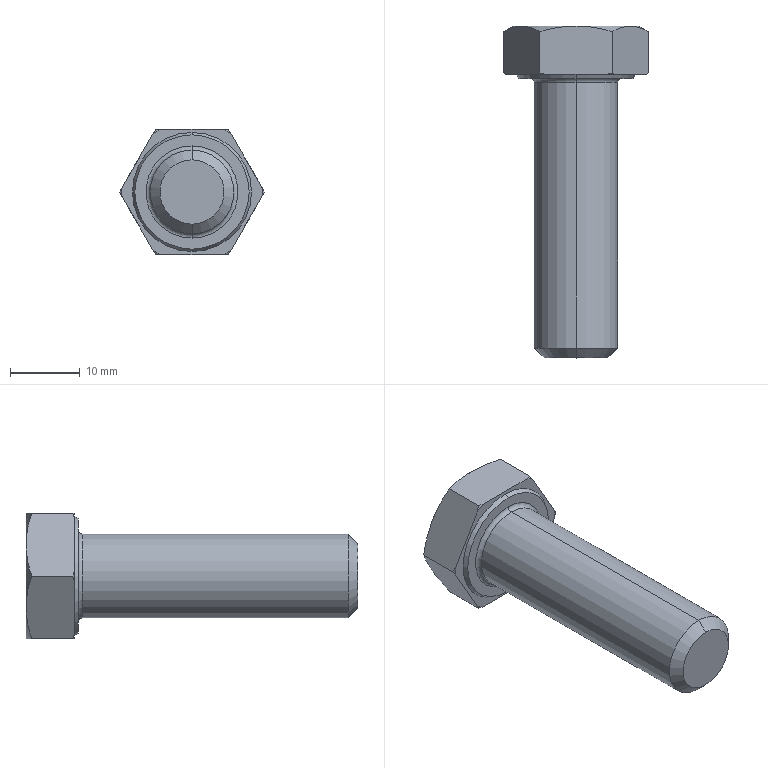Component | SolidWorks | GB_T5781-2000[HexHeadBoltFullThreadGradeCM12_40]-1 | 1 solid | 30 faces | box 20.78 x 47.5 x 18 mm | volume 6554 mm3 | cone 16 | plane 10 | cylinder 2 | torus 2 | commonest cylinder face diameters 12 x2
build123d program:
from build123d import *

# Parameters (mm, degrees)
BASE_EXTRUDE_DEPTH = 7.5
CHAMFER_2_SIZE     = 1.4


with BuildPart() as part:
    # Sketch1 → Base-Extrude (new body)
    with BuildSketch(Plane(origin=(0, 0, 0), x_dir=(0, 0, -1), z_dir=(1, 0, 0))):
        Polygon((9, 5.196), (9, -5.196), (0, -10.392), (-9, -5.196), (-9, 5.196), (0, 10.392), align=None)
    extrude(amount=BASE_EXTRUDE_DEPTH)

    # Sketch2 → Revolve1 (revolve)
    with BuildSketch(Plane.XY, mode=Mode.PRIVATE) as revolve1_sk:
        Polygon((0, 0), (47.5, 0), (47.5, 4.484), (47.5, 6), (7.5, 6), (0, 6), align=None)
    revolve(revolve1_sk.sketch.rotate(Axis((0, 0, 0), (-1, 0, 0)), 90), axis=Axis((0, 0, 0), (-1, 0, 0)))

    # Sketch3 → Cut-Revolve1 (revolve, cut)
    with BuildSketch(Plane.XY):
        Polygon((0, 9), (3.691, 15.392), (3.691, 20.392), (-10, 20.392), (-10, 9), align=None)
    revolve(axis=Axis((0, 0, 0), (1, 0, 0)), mode=Mode.SUBTRACT)

    # Sketch5 → Cut-Revolve2 (revolve, cut)
    with BuildSketch(Plane.XY):
        Polygon((7.5, 9), (3.809, 15.392), (3.809, 20.392), (13.809, 20.392), (13.809, 9), align=None)
    revolve(axis=Axis((0, 0, 0), (1, 0, 0)), mode=Mode.SUBTRACT)

    # Sketch4 → Cut-Revolve3 (revolve, cut)
    with BuildSketch(Plane.XY, mode=Mode.PRIVATE) as cut_revolve3_sk:
        Polygon((7.5, 8.177), (6.9, 8.524), (6.9, 20.392), (7.5, 20.392), align=None)
    revolve(cut_revolve3_sk.sketch.rotate(Axis((0, 0, 0), (1, 0, 0)), 90), axis=Axis((0, 0, 0), (1, 0, 0)), mode=Mode.SUBTRACT)

    # Chamfer 2
    chamfer_2_edges = [part.edges().sort_by_distance(p)[0] for p in [
        (47.5, 0, 6),
    ]]
    chamfer(chamfer_2_edges, length=CHAMFER_2_SIZE)

    # Sketch9 → Revolve1_2 (revolve)
    with BuildSketch(Plane.XY, mode=Mode.PRIVATE) as revolve1_2_sk:
        with BuildLine():
            Line((7.5, 6.6), (7.5, 6))
            Line((7.5, 6), (8.1, 6))
            ThreePointArc((8.1, 6), (7.676, 6.176), (7.5, 6.6))
        make_face()
    revolve(revolve1_2_sk.sketch.rotate(Axis((0, 0, 0), (1, 0, 0)), 90), axis=Axis((0, 0, 0), (1, 0, 0)))


solid = part.part

# Placed as in the assembly
solid = solid.moved(Location((110, 17.5, 125), (0, 0, -90)))
STEP:
#1=COLOUR_RGB('',0.7922,0.8196,0.9333);
#2=FILL_AREA_STYLE_COLOUR('',#1);
#3=FILL_AREA_STYLE('',(#2));
#4=SURFACE_STYLE_FILL_AREA(#3);
#5=SURFACE_SIDE_STYLE('',(#4));
#6=SURFACE_STYLE_USAGE(.BOTH.,#5);
#7=PRESENTATION_STYLE_ASSIGNMENT((#6));
#8=CARTESIAN_POINT('',(4.331,0.3701,5.157));
#9=VERTEX_POINT('',#8);
#10=CARTESIAN_POINT('',(4.331,0.3701,4.685));
#11=VERTEX_POINT('',#10);
#12=CARTESIAN_POINT('',(4.331,0.3701,4.921));
#13=DIRECTION('',(-0.,1.,0.));
#14=DIRECTION('',(0.,0.,1.));
#15=AXIS2_PLACEMENT_3D('',#12,#13,#14);
#16=CIRCLE('',#15,0.2362);
#17=EDGE_CURVE('',#9,#11,#16,.T.);
#18=ORIENTED_EDGE('',*,*,#17,.F.);
#19=CARTESIAN_POINT('',(4.331,-1.126,5.157));
#20=VERTEX_POINT('',#19);
#21=CARTESIAN_POINT('',(4.331,0.689,5.157));
#22=DIRECTION('',(0.,-1.,0.));
#23=VECTOR('',#22,39.37);
#24=LINE('',#21,#23);
#25=EDGE_CURVE('',#9,#20,#24,.T.);
#26=ORIENTED_EDGE('',*,*,#25,.T.);
#27=CARTESIAN_POINT('',(4.331,-1.126,4.685));
#28=VERTEX_POINT('',#27);
#29=CARTESIAN_POINT('',(4.331,-1.126,4.921));
#30=DIRECTION('',(-0.,1.,0.));
#31=DIRECTION('',(0.,0.,-1.));
#32=AXIS2_PLACEMENT_3D('',#29,#30,#31);
#33=CIRCLE('',#32,0.2362);
#34=EDGE_CURVE('',#20,#28,#33,.T.);
#35=ORIENTED_EDGE('',*,*,#34,.T.);
#36=CARTESIAN_POINT('',(4.331,0.689,4.685));
#37=DIRECTION('',(0.,-1.,0.));
#38=VECTOR('',#37,39.37);
#39=LINE('',#36,#38);
#40=EDGE_CURVE('',#11,#28,#39,.T.);
#41=ORIENTED_EDGE('',*,*,#40,.F.);
#42=EDGE_LOOP('',(#18,#26,#35,#41));
#43=FACE_OUTER_BOUND('',#42,.T.);
#44=CARTESIAN_POINT('',(4.331,0.689,4.921));
#45=DIRECTION('',(0.,-1.,0.));
#46=DIRECTION('',(0.,0.,-1.));
#47=AXIS2_PLACEMENT_3D('',#44,#45,#46);
#48=CYLINDRICAL_SURFACE('',#47,0.2362);
#49=ADVANCED_FACE('',(#43),#48,.T.);
#50=CARTESIAN_POINT('',(4.331,-1.181,4.74));
#51=VERTEX_POINT('',#50);
#52=CARTESIAN_POINT('',(4.331,-1.181,5.102));
#53=VERTEX_POINT('',#52);
#54=CARTESIAN_POINT('',(4.331,-1.181,4.921));
#55=DIRECTION('',(0.,-1.,0.));
#56=DIRECTION('',(0.,0.,-1.));
#57=AXIS2_PLACEMENT_3D('',#54,#55,#56);
#58=CIRCLE('',#57,0.1811);
#59=EDGE_CURVE('',#51,#53,#58,.T.);
#60=ORIENTED_EDGE('',*,*,#59,.F.);
#61=CARTESIAN_POINT('',(4.331,-1.181,4.74));
#62=DIRECTION('',(-0.,0.7071,-0.7071));
#63=VECTOR('',#62,39.37);
#64=LINE('',#61,#63);
#65=EDGE_CURVE('',#51,#28,#64,.T.);
#66=ORIENTED_EDGE('',*,*,#65,.T.);
#67=ORIENTED_EDGE('',*,*,#34,.F.);
#68=CARTESIAN_POINT('',(4.331,-1.181,5.102));
#69=DIRECTION('',(-0.,0.7071,0.7071));
#70=VECTOR('',#69,39.37);
#71=LINE('',#68,#70);
#72=EDGE_CURVE('',#53,#20,#71,.T.);
#73=ORIENTED_EDGE('',*,*,#72,.F.);
#74=EDGE_LOOP('',(#60,#66,#67,#73));
#75=FACE_OUTER_BOUND('',#74,.T.);
#76=CARTESIAN_POINT('',(4.331,-1.181,4.921));
#77=DIRECTION('',(-0.,1.,0.));
#78=DIRECTION('',(0.,0.,1.));
#79=AXIS2_PLACEMENT_3D('',#76,#77,#78);
#80=CONICAL_SURFACE('',#79,0.1811,0.7854);
#81=ADVANCED_FACE('',(#75),#80,.T.);
#82=CARTESIAN_POINT('',(4.331,0.3937,4.661));
#83=VERTEX_POINT('',#82);
#84=CARTESIAN_POINT('',(4.331,0.3937,5.181));
#85=VERTEX_POINT('',#84);
#86=CARTESIAN_POINT('',(4.331,0.3937,4.921));
#87=DIRECTION('',(-0.,1.,0.));
#88=DIRECTION('',(0.,0.,1.));
#89=AXIS2_PLACEMENT_3D('',#86,#87,#88);
#90=CIRCLE('',#89,0.2598);
#91=EDGE_CURVE('',#83,#85,#90,.T.);
#92=ORIENTED_EDGE('',*,*,#91,.F.);
#93=CARTESIAN_POINT('',(4.331,0.3701,4.661));
#94=DIRECTION('',(1.,0.,0.));
#95=DIRECTION('',(0.,1.,0.));
#96=AXIS2_PLACEMENT_3D('',#93,#94,#95);
#97=CIRCLE('',#96,0.02362);
#98=EDGE_CURVE('',#83,#11,#97,.T.);
#99=ORIENTED_EDGE('',*,*,#98,.T.);
#100=CARTESIAN_POINT('',(4.331,0.3701,4.921));
#101=DIRECTION('',(-0.,1.,0.));
#102=DIRECTION('',(0.,0.,1.));
#103=AXIS2_PLACEMENT_3D('',#100,#101,#102);
#104=CIRCLE('',#103,0.2362);
#105=EDGE_CURVE('',#11,#9,#104,.T.);
#106=ORIENTED_EDGE('',*,*,#105,.T.);
#107=CARTESIAN_POINT('',(4.331,0.3701,5.181));
#108=DIRECTION('',(-1.,-0.,0.));
#109=DIRECTION('',(0.,-1.,0.));
#110=AXIS2_PLACEMENT_3D('',#107,#108,#109);
#111=CIRCLE('',#110,0.02362);
#112=EDGE_CURVE('',#85,#9,#111,.T.);
#113=ORIENTED_EDGE('',*,*,#112,.F.);
#114=EDGE_LOOP('',(#92,#99,#106,#113));
#115=FACE_OUTER_BOUND('',#114,.T.);
#116=CARTESIAN_POINT('',(4.331,0.3701,4.921));
#117=DIRECTION('',(-0.,1.,0.));
#118=DIRECTION('',(0.,0.,1.));
#119=AXIS2_PLACEMENT_3D('',#116,#117,#118);
#120=TOROIDAL_SURFACE('',#119,0.2598,0.02362);
#121=ADVANCED_FACE('',(#115),#120,.F.);
#122=CARTESIAN_POINT('',(4.331,0.3937,5.243));
#123=VERTEX_POINT('',#122);
#124=CARTESIAN_POINT('',(4.331,0.3937,4.599));
#125=VERTEX_POINT('',#124);
#126=CARTESIAN_POINT('',(4.331,0.3937,4.921));
#127=DIRECTION('',(-0.,1.,0.));
#128=DIRECTION('',(0.,0.,1.));
#129=AXIS2_PLACEMENT_3D('',#126,#127,#128);
#130=CIRCLE('',#129,0.3219);
#131=EDGE_CURVE('',#123,#125,#130,.T.);
#132=ORIENTED_EDGE('',*,*,#131,.T.);
#133=CARTESIAN_POINT('',(4.331,0.4173,4.586));
#134=VERTEX_POINT('',#133);
#135=CARTESIAN_POINT('',(4.331,0.4173,4.586));
#136=DIRECTION('',(-0.,0.866,-0.5));
#137=VECTOR('',#136,39.37);
#138=LINE('',#135,#137);
#139=EDGE_CURVE('',#125,#134,#138,.T.);
#140=ORIENTED_EDGE('',*,*,#139,.T.);
#141=CARTESIAN_POINT('',(4.331,0.4173,5.257));
#142=VERTEX_POINT('',#141);
#143=CARTESIAN_POINT('',(4.331,0.4173,4.921));
#144=DIRECTION('',(-0.,1.,0.));
#145=DIRECTION('',(0.,0.,1.));
#146=AXIS2_PLACEMENT_3D('',#143,#144,#145);
#147=CIRCLE('',#146,0.3356);
#148=EDGE_CURVE('',#142,#134,#147,.T.);
#149=ORIENTED_EDGE('',*,*,#148,.F.);
#150=CARTESIAN_POINT('',(4.331,0.4173,5.257));
#151=DIRECTION('',(-0.,0.866,0.5));
#152=VECTOR('',#151,39.37);
#153=LINE('',#150,#152);
#154=EDGE_CURVE('',#123,#142,#153,.T.);
#155=ORIENTED_EDGE('',*,*,#154,.F.);
#156=EDGE_LOOP('',(#132,#140,#149,#155));
#157=FACE_OUTER_BOUND('',#156,.T.);
#158=CARTESIAN_POINT('',(4.331,0.4173,4.921));
#159=DIRECTION('',(-0.,1.,0.));
#160=DIRECTION('',(0.,0.,1.));
#161=AXIS2_PLACEMENT_3D('',#158,#159,#160);
#162=CONICAL_SURFACE('',#161,0.3356,0.5236);
#163=ADVANCED_FACE('',(#157),#162,.T.);
#164=ORIENTED_EDGE('',*,*,#131,.F.);
#165=CARTESIAN_POINT('',(4.331,0.3937,4.921));
#166=DIRECTION('',(-0.,1.,0.));
#167=DIRECTION('',(0.,0.,1.));
#168=AXIS2_PLACEMENT_3D('',#165,#166,#167);
#169=CIRCLE('',#168,0.3219);
#170=EDGE_CURVE('',#125,#123,#169,.T.);
#171=ORIENTED_EDGE('',*,*,#170,.F.);
#172=EDGE_LOOP('',(#164,#171));
#173=FACE_OUTER_BOUND('',#172,.T.);
#174=CARTESIAN_POINT('',(4.331,0.3937,4.921));
#175=DIRECTION('',(-0.,1.,0.));
#176=DIRECTION('',(0.,0.,1.));
#177=AXIS2_PLACEMENT_3D('',#174,#175,#176);
#178=CIRCLE('',#177,0.2598);
#179=EDGE_CURVE('',#85,#83,#178,.T.);
#180=ORIENTED_EDGE('',*,*,#179,.T.);
#181=ORIENTED_EDGE('',*,*,#91,.T.);
#182=EDGE_LOOP('',(#180,#181));
#183=FACE_BOUND('',#182,.T.);
#184=CARTESIAN_POINT('',(4.74,0.3937,4.921));
#185=DIRECTION('',(0.,-1.,0.));
#186=DIRECTION('',(0.,0.,-1.));
#187=AXIS2_PLACEMENT_3D('',#184,#185,#186);
#188=PLANE('',#187);
#189=ADVANCED_FACE('',(#173,#183),#188,.T.);
#190=CARTESIAN_POINT('',(4.55,0.4173,4.592));
#191=VERTEX_POINT('',#190);
#192=CARTESIAN_POINT('',(4.725,0.4173,4.896));
#193=VERTEX_POINT('',#192);
#194=CARTESIAN_POINT('',(4.535,0.4173,4.567));
#195=DIRECTION('',(0.5,0.,0.866));
#196=VECTOR('',#195,39.37);
#197=LINE('',#194,#196);
#198=EDGE_CURVE('',#191,#193,#197,.T.);
#199=ORIENTED_EDGE('',*,*,#198,.F.);
#200=CARTESIAN_POINT('',(4.535,0.4253,4.567));
#201=VERTEX_POINT('',#200);
#202=CARTESIAN_POINT('',(4.535,0.4253,4.567));
#203=CARTESIAN_POINT('',(4.54,0.4225,4.575));
#204=CARTESIAN_POINT('',(4.545,0.4198,4.584));
#205=CARTESIAN_POINT('',(4.55,0.4173,4.592));
#206=B_SPLINE_CURVE_WITH_KNOTS('',3,(#202,#203,#204,#205),.UNSPECIFIED.,.F.,.F.,(4,4),(0.00000024,0.0007696),.UNSPECIFIED.);
#207=EDGE_CURVE('',#201,#191,#206,.T.);
#208=ORIENTED_EDGE('',*,*,#207,.F.);
#209=CARTESIAN_POINT('',(4.535,0.6573,4.567));
#210=VERTEX_POINT('',#209);
#211=CARTESIAN_POINT('',(4.535,0.3937,4.567));
#212=DIRECTION('',(-0.,1.,0.));
#213=VECTOR('',#212,39.37);
#214=LINE('',#211,#213);
#215=EDGE_CURVE('',#201,#210,#214,.T.);
#216=ORIENTED_EDGE('',*,*,#215,.T.);
#217=CARTESIAN_POINT('',(4.638,0.689,4.744));
#218=VERTEX_POINT('',#217);
#219=CARTESIAN_POINT('',(4.638,0.689,4.744));
#220=CARTESIAN_POINT('',(4.629,0.689,4.729));
#221=CARTESIAN_POINT('',(4.62,0.6882,4.714));
#222=CARTESIAN_POINT('',(4.603,0.6853,4.684));
#223=CARTESIAN_POINT('',(4.594,0.6832,4.669));
#224=CARTESIAN_POINT('',(4.569,0.6749,4.625));
#225=CARTESIAN_POINT('',(4.552,0.667,4.596));
#226=CARTESIAN_POINT('',(4.535,0.6573,4.567));
#227=B_SPLINE_CURVE_WITH_KNOTS('',3,(#219,#220,#221,#222,#223,#224,#225,#226),.UNSPECIFIED.,.F.,.F.,(4,2,2,4),(0.005258,0.006567,0.007877,0.0105),.UNSPECIFIED.);
#228=EDGE_CURVE('',#218,#210,#227,.T.);
#229=ORIENTED_EDGE('',*,*,#228,.F.);
#230=CARTESIAN_POINT('',(4.74,0.6573,4.921));
#231=VERTEX_POINT('',#230);
#232=CARTESIAN_POINT('',(4.74,0.6573,4.921));
#233=CARTESIAN_POINT('',(4.723,0.667,4.892));
#234=CARTESIAN_POINT('',(4.706,0.6749,4.863));
#235=CARTESIAN_POINT('',(4.672,0.686,4.804));
#236=CARTESIAN_POINT('',(4.655,0.689,4.774));
#237=CARTESIAN_POINT('',(4.638,0.689,4.744));
#238=B_SPLINE_CURVE_WITH_KNOTS('',3,(#232,#233,#234,#235,#236,#237),.UNSPECIFIED.,.F.,.F.,(4,2,4),(0.00000024,0.002629,0.005258),.UNSPECIFIED.);
#239=EDGE_CURVE('',#231,#218,#238,.T.);
#240=ORIENTED_EDGE('',*,*,#239,.F.);
#241=CARTESIAN_POINT('',(4.74,0.4253,4.921));
#242=VERTEX_POINT('',#241);
#243=CARTESIAN_POINT('',(4.74,0.3937,4.921));
#244=DIRECTION('',(-0.,1.,0.));
#245=VECTOR('',#244,39.37);
#246=LINE('',#243,#245);
#247=EDGE_CURVE('',#242,#231,#246,.T.);
#248=ORIENTED_EDGE('',*,*,#247,.F.);
#249=CARTESIAN_POINT('',(4.725,0.4173,4.896));
#250=CARTESIAN_POINT('',(4.73,0.4198,4.904));
#251=CARTESIAN_POINT('',(4.735,0.4225,4.913));
#252=CARTESIAN_POINT('',(4.74,0.4253,4.921));
#253=B_SPLINE_CURVE_WITH_KNOTS('',3,(#249,#250,#251,#252),.UNSPECIFIED.,.F.,.F.,(4,4),(0.009728,0.0105),.UNSPECIFIED.);
#254=EDGE_CURVE('',#193,#242,#253,.T.);
#255=ORIENTED_EDGE('',*,*,#254,.F.);
#256=EDGE_LOOP('',(#199,#208,#216,#229,#240,#248,#255));
#257=FACE_OUTER_BOUND('',#256,.T.);
#258=CARTESIAN_POINT('',(4.535,0.3937,4.567));
#259=DIRECTION('',(-0.866,-0.,0.5));
#260=DIRECTION('',(-0.5,-0.,-0.866));
#261=AXIS2_PLACEMENT_3D('',#258,#259,#260);
#262=PLANE('',#261);
#263=ADVANCED_FACE('',(#257),#262,.F.);
#264=CARTESIAN_POINT('',(4.725,0.4173,4.947));
#265=VERTEX_POINT('',#264);
#266=CARTESIAN_POINT('',(4.55,0.4173,5.25));
#267=VERTEX_POINT('',#266);
#268=CARTESIAN_POINT('',(4.74,0.4173,4.921));
#269=DIRECTION('',(-0.5,-0.,0.866));
#270=VECTOR('',#269,39.37);
#271=LINE('',#268,#270);
#272=EDGE_CURVE('',#265,#267,#271,.T.);
#273=ORIENTED_EDGE('',*,*,#272,.F.);
#274=CARTESIAN_POINT('',(4.74,0.4253,4.921));
#275=CARTESIAN_POINT('',(4.735,0.4225,4.93));
#276=CARTESIAN_POINT('',(4.73,0.4198,4.938));
#277=CARTESIAN_POINT('',(4.725,0.4173,4.947));
#278=B_SPLINE_CURVE_WITH_KNOTS('',3,(#274,#275,#276,#277),.UNSPECIFIED.,.F.,.F.,(4,4),(0.00000024,0.0007696),.UNSPECIFIED.);
#279=EDGE_CURVE('',#242,#265,#278,.T.);
#280=ORIENTED_EDGE('',*,*,#279,.F.);
#281=ORIENTED_EDGE('',*,*,#247,.T.);
#282=CARTESIAN_POINT('',(4.638,0.689,5.098));
#283=VERTEX_POINT('',#282);
#284=CARTESIAN_POINT('',(4.638,0.689,5.098));
#285=CARTESIAN_POINT('',(4.646,0.689,5.083));
#286=CARTESIAN_POINT('',(4.655,0.6882,5.068));
#287=CARTESIAN_POINT('',(4.672,0.6853,5.038));
#288=CARTESIAN_POINT('',(4.681,0.6832,5.024));
#289=CARTESIAN_POINT('',(4.706,0.6749,4.979));
#290=CARTESIAN_POINT('',(4.723,0.667,4.95));
#291=CARTESIAN_POINT('',(4.74,0.6573,4.921));
#292=B_SPLINE_CURVE_WITH_KNOTS('',3,(#284,#285,#286,#287,#288,#289,#290,#291),.UNSPECIFIED.,.F.,.F.,(4,2,2,4),(0.005258,0.006567,0.007877,0.0105),.UNSPECIFIED.);
#293=EDGE_CURVE('',#283,#231,#292,.T.);
#294=ORIENTED_EDGE('',*,*,#293,.F.);
#295=CARTESIAN_POINT('',(4.535,0.6573,5.276));
#296=VERTEX_POINT('',#295);
#297=CARTESIAN_POINT('',(4.535,0.6573,5.276));
#298=CARTESIAN_POINT('',(4.552,0.667,5.247));
#299=CARTESIAN_POINT('',(4.569,0.6749,5.217));
#300=CARTESIAN_POINT('',(4.603,0.686,5.158));
#301=CARTESIAN_POINT('',(4.62,0.689,5.129));
#302=CARTESIAN_POINT('',(4.638,0.689,5.098));
#303=B_SPLINE_CURVE_WITH_KNOTS('',3,(#297,#298,#299,#300,#301,#302),.UNSPECIFIED.,.F.,.F.,(4,2,4),(0.00000024,0.002629,0.005258),.UNSPECIFIED.);
#304=EDGE_CURVE('',#296,#283,#303,.T.);
#305=ORIENTED_EDGE('',*,*,#304,.F.);
#306=CARTESIAN_POINT('',(4.535,0.4253,5.276));
#307=VERTEX_POINT('',#306);
#308=CARTESIAN_POINT('',(4.535,0.3937,5.276));
#309=DIRECTION('',(-0.,1.,0.));
#310=VECTOR('',#309,39.37);
#311=LINE('',#308,#310);
#312=EDGE_CURVE('',#307,#296,#311,.T.);
#313=ORIENTED_EDGE('',*,*,#312,.F.);
#314=CARTESIAN_POINT('',(4.55,0.4173,5.25));
#315=CARTESIAN_POINT('',(4.545,0.4198,5.259));
#316=CARTESIAN_POINT('',(4.54,0.4225,5.267));
#317=CARTESIAN_POINT('',(4.535,0.4253,5.276));
#318=B_SPLINE_CURVE_WITH_KNOTS('',3,(#314,#315,#316,#317),.UNSPECIFIED.,.F.,.F.,(4,4),(0.009728,0.0105),.UNSPECIFIED.);
#319=EDGE_CURVE('',#267,#307,#318,.T.);
#320=ORIENTED_EDGE('',*,*,#319,.F.);
#321=EDGE_LOOP('',(#273,#280,#281,#294,#305,#313,#320));
#322=FACE_OUTER_BOUND('',#321,.T.);
#323=CARTESIAN_POINT('',(4.74,0.3937,4.921));
#324=DIRECTION('',(-0.866,-0.,-0.5));
#325=DIRECTION('',(0.5,0.,-0.866));
#326=AXIS2_PLACEMENT_3D('',#323,#324,#325);
#327=PLANE('',#326);
#328=ADVANCED_FACE('',(#322),#327,.F.);
#329=CARTESIAN_POINT('',(4.506,0.4173,5.276));
#330=VERTEX_POINT('',#329);
#331=CARTESIAN_POINT('',(4.156,0.4173,5.276));
#332=VERTEX_POINT('',#331);
#333=CARTESIAN_POINT('',(4.535,0.4173,5.276));
#334=DIRECTION('',(-1.,-0.,-0.));
#335=VECTOR('',#334,39.37);
#336=LINE('',#333,#335);
#337=EDGE_CURVE('',#330,#332,#336,.T.);
#338=ORIENTED_EDGE('',*,*,#337,.F.);
#339=CARTESIAN_POINT('',(4.535,0.4253,5.276));
#340=CARTESIAN_POINT('',(4.526,0.4225,5.276));
#341=CARTESIAN_POINT('',(4.516,0.4198,5.276));
#342=CARTESIAN_POINT('',(4.506,0.4173,5.276));
#343=B_SPLINE_CURVE_WITH_KNOTS('',3,(#339,#340,#341,#342),.UNSPECIFIED.,.F.,.F.,(4,4),(0.02519,0.02597),.UNSPECIFIED.);
#344=EDGE_CURVE('',#307,#330,#343,.T.);
#345=ORIENTED_EDGE('',*,*,#344,.F.);
#346=ORIENTED_EDGE('',*,*,#312,.T.);
#347=CARTESIAN_POINT('',(4.331,0.689,5.276));
#348=VERTEX_POINT('',#347);
#349=CARTESIAN_POINT('',(4.331,0.689,5.276));
#350=CARTESIAN_POINT('',(4.348,0.689,5.276));
#351=CARTESIAN_POINT('',(4.365,0.6882,5.276));
#352=CARTESIAN_POINT('',(4.4,0.6853,5.276));
#353=CARTESIAN_POINT('',(4.417,0.6831,5.276));
#354=CARTESIAN_POINT('',(4.469,0.6748,5.276));
#355=CARTESIAN_POINT('',(4.502,0.6669,5.276));
#356=CARTESIAN_POINT('',(4.535,0.6573,5.276));
#357=B_SPLINE_CURVE_WITH_KNOTS('',3,(#349,#350,#351,#352,#353,#354,#355,#356),.UNSPECIFIED.,.F.,.F.,(4,2,2,4),(0.01498,0.0163,0.01761,0.02025),.UNSPECIFIED.);
#358=EDGE_CURVE('',#348,#296,#357,.T.);
#359=ORIENTED_EDGE('',*,*,#358,.F.);
#360=CARTESIAN_POINT('',(4.126,0.6573,5.276));
#361=VERTEX_POINT('',#360);
#362=CARTESIAN_POINT('',(4.126,0.6573,5.276));
#363=CARTESIAN_POINT('',(4.159,0.6669,5.276));
#364=CARTESIAN_POINT('',(4.194,0.675,5.276));
#365=CARTESIAN_POINT('',(4.262,0.686,5.276));
#366=CARTESIAN_POINT('',(4.296,0.689,5.276));
#367=CARTESIAN_POINT('',(4.331,0.689,5.276));
#368=B_SPLINE_CURVE_WITH_KNOTS('',3,(#362,#363,#364,#365,#366,#367),.UNSPECIFIED.,.F.,.F.,(4,2,4),(0.00972,0.01235,0.01498),.UNSPECIFIED.);
#369=EDGE_CURVE('',#361,#348,#368,.T.);
#370=ORIENTED_EDGE('',*,*,#369,.F.);
#371=CARTESIAN_POINT('',(4.126,0.4253,5.276));
#372=VERTEX_POINT('',#371);
#373=CARTESIAN_POINT('',(4.126,0.3937,5.276));
#374=DIRECTION('',(-0.,1.,0.));
#375=VECTOR('',#374,39.37);
#376=LINE('',#373,#375);
#377=EDGE_CURVE('',#372,#361,#376,.T.);
#378=ORIENTED_EDGE('',*,*,#377,.F.);
#379=CARTESIAN_POINT('',(4.156,0.4173,5.276));
#380=CARTESIAN_POINT('',(4.146,0.4198,5.276));
#381=CARTESIAN_POINT('',(4.136,0.4225,5.276));
#382=CARTESIAN_POINT('',(4.126,0.4253,5.276));
#383=B_SPLINE_CURVE_WITH_KNOTS('',3,(#379,#380,#381,#382),.UNSPECIFIED.,.F.,.F.,(4,4),(0.03494,0.03571),.UNSPECIFIED.);
#384=EDGE_CURVE('',#332,#372,#383,.T.);
#385=ORIENTED_EDGE('',*,*,#384,.F.);
#386=EDGE_LOOP('',(#338,#345,#346,#359,#370,#378,#385));
#387=FACE_OUTER_BOUND('',#386,.T.);
#388=CARTESIAN_POINT('',(4.535,0.3937,5.276));
#389=DIRECTION('',(0.,0.,-1.));
#390=DIRECTION('',(1.,0.,0.));
#391=AXIS2_PLACEMENT_3D('',#388,#389,#390);
#392=PLANE('',#391);
#393=ADVANCED_FACE('',(#387),#392,.F.);
#394=CARTESIAN_POINT('',(4.111,0.4173,5.25));
#395=VERTEX_POINT('',#394);
#396=CARTESIAN_POINT('',(3.936,0.4173,4.947));
#397=VERTEX_POINT('',#396);
#398=CARTESIAN_POINT('',(3.922,0.4173,4.921));
#399=DIRECTION('',(-0.5,-0.,-0.866));
#400=VECTOR('',#399,39.37);
#401=LINE('',#398,#400);
#402=EDGE_CURVE('',#395,#397,#401,.T.);
#403=ORIENTED_EDGE('',*,*,#402,.F.);
#404=CARTESIAN_POINT('',(4.126,0.4253,5.276));
#405=CARTESIAN_POINT('',(4.121,0.4225,5.267));
#406=CARTESIAN_POINT('',(4.116,0.4198,5.259));
#407=CARTESIAN_POINT('',(4.111,0.4173,5.25));
#408=B_SPLINE_CURVE_WITH_KNOTS('',3,(#404,#405,#406,#407),.UNSPECIFIED.,.F.,.F.,(4,4),(0.00000024,0.0007696),.UNSPECIFIED.);
#409=EDGE_CURVE('',#372,#395,#408,.T.);
#410=ORIENTED_EDGE('',*,*,#409,.F.);
#411=ORIENTED_EDGE('',*,*,#377,.T.);
#412=CARTESIAN_POINT('',(4.024,0.689,5.098));
#413=VERTEX_POINT('',#412);
#414=CARTESIAN_POINT('',(4.024,0.689,5.098));
#415=CARTESIAN_POINT('',(4.033,0.689,5.113));
#416=CARTESIAN_POINT('',(4.041,0.6882,5.129));
#417=CARTESIAN_POINT('',(4.058,0.6853,5.158));
#418=CARTESIAN_POINT('',(4.067,0.6832,5.173));
#419=CARTESIAN_POINT('',(4.093,0.6749,5.218));
#420=CARTESIAN_POINT('',(4.109,0.667,5.247));
#421=CARTESIAN_POINT('',(4.126,0.6573,5.276));
#422=B_SPLINE_CURVE_WITH_KNOTS('',3,(#414,#415,#416,#417,#418,#419,#420,#421),.UNSPECIFIED.,.F.,.F.,(4,2,2,4),(0.005258,0.006567,0.007877,0.0105),.UNSPECIFIED.);
#423=EDGE_CURVE('',#413,#361,#422,.T.);
#424=ORIENTED_EDGE('',*,*,#423,.F.);
#425=CARTESIAN_POINT('',(3.922,0.6573,4.921));
#426=VERTEX_POINT('',#425);
#427=CARTESIAN_POINT('',(3.922,0.6573,4.921));
#428=CARTESIAN_POINT('',(3.938,0.667,4.95));
#429=CARTESIAN_POINT('',(3.955,0.6749,4.979));
#430=CARTESIAN_POINT('',(3.989,0.686,5.038));
#431=CARTESIAN_POINT('',(4.006,0.689,5.068));
#432=CARTESIAN_POINT('',(4.024,0.689,5.098));
#433=B_SPLINE_CURVE_WITH_KNOTS('',3,(#427,#428,#429,#430,#431,#432),.UNSPECIFIED.,.F.,.F.,(4,2,4),(0.00000024,0.002629,0.005258),.UNSPECIFIED.);
#434=EDGE_CURVE('',#426,#413,#433,.T.);
#435=ORIENTED_EDGE('',*,*,#434,.F.);
#436=CARTESIAN_POINT('',(3.922,0.4253,4.921));
#437=VERTEX_POINT('',#436);
#438=CARTESIAN_POINT('',(3.922,0.3937,4.921));
#439=DIRECTION('',(-0.,1.,0.));
#440=VECTOR('',#439,39.37);
#441=LINE('',#438,#440);
#442=EDGE_CURVE('',#437,#426,#441,.T.);
#443=ORIENTED_EDGE('',*,*,#442,.F.);
#444=CARTESIAN_POINT('',(3.936,0.4173,4.947));
#445=CARTESIAN_POINT('',(3.931,0.4198,4.938));
#446=CARTESIAN_POINT('',(3.926,0.4225,4.93));
#447=CARTESIAN_POINT('',(3.922,0.4253,4.921));
#448=B_SPLINE_CURVE_WITH_KNOTS('',3,(#444,#445,#446,#447),.UNSPECIFIED.,.F.,.F.,(4,4),(0.009728,0.0105),.UNSPECIFIED.);
#449=EDGE_CURVE('',#397,#437,#448,.T.);
#450=ORIENTED_EDGE('',*,*,#449,.F.);
#451=EDGE_LOOP('',(#403,#410,#411,#424,#435,#443,#450));
#452=FACE_OUTER_BOUND('',#451,.T.);
#453=CARTESIAN_POINT('',(3.922,0.3937,4.921));
#454=DIRECTION('',(0.866,0.,-0.5));
#455=DIRECTION('',(0.5,0.,0.866));
#456=AXIS2_PLACEMENT_3D('',#453,#454,#455);
#457=PLANE('',#456);
#458=ADVANCED_FACE('',(#452),#457,.F.);
#459=CARTESIAN_POINT('',(3.936,0.4173,4.896));
#460=VERTEX_POINT('',#459);
#461=CARTESIAN_POINT('',(4.111,0.4173,4.592));
#462=VERTEX_POINT('',#461);
#463=CARTESIAN_POINT('',(4.126,0.4173,4.567));
#464=DIRECTION('',(0.5,0.,-0.866));
#465=VECTOR('',#464,39.37);
#466=LINE('',#463,#465);
#467=EDGE_CURVE('',#460,#462,#466,.T.);
#468=ORIENTED_EDGE('',*,*,#467,.F.);
#469=CARTESIAN_POINT('',(3.922,0.4253,4.921));
#470=CARTESIAN_POINT('',(3.926,0.4225,4.913));
#471=CARTESIAN_POINT('',(3.931,0.4198,4.904));
#472=CARTESIAN_POINT('',(3.936,0.4173,4.896));
#473=B_SPLINE_CURVE_WITH_KNOTS('',3,(#469,#470,#471,#472),.UNSPECIFIED.,.F.,.F.,(4,4),(0.00000024,0.0007696),.UNSPECIFIED.);
#474=EDGE_CURVE('',#437,#460,#473,.T.);
#475=ORIENTED_EDGE('',*,*,#474,.F.);
#476=ORIENTED_EDGE('',*,*,#442,.T.);
#477=CARTESIAN_POINT('',(4.024,0.689,4.744));
#478=VERTEX_POINT('',#477);
#479=CARTESIAN_POINT('',(4.024,0.689,4.744));
#480=CARTESIAN_POINT('',(4.015,0.689,4.759));
#481=CARTESIAN_POINT('',(4.006,0.6882,4.774));
#482=CARTESIAN_POINT('',(3.989,0.6853,4.804));
#483=CARTESIAN_POINT('',(3.981,0.6832,4.819));
#484=CARTESIAN_POINT('',(3.955,0.6749,4.863));
#485=CARTESIAN_POINT('',(3.938,0.667,4.892));
#486=CARTESIAN_POINT('',(3.922,0.6573,4.921));
#487=B_SPLINE_CURVE_WITH_KNOTS('',3,(#479,#480,#481,#482,#483,#484,#485,#486),.UNSPECIFIED.,.F.,.F.,(4,2,2,4),(0.005258,0.006567,0.007877,0.0105),.UNSPECIFIED.);
#488=EDGE_CURVE('',#478,#426,#487,.T.);
#489=ORIENTED_EDGE('',*,*,#488,.F.);
#490=CARTESIAN_POINT('',(4.126,0.6573,4.567));
#491=VERTEX_POINT('',#490);
#492=CARTESIAN_POINT('',(4.126,0.6573,4.567));
#493=CARTESIAN_POINT('',(4.109,0.667,4.596));
#494=CARTESIAN_POINT('',(4.093,0.6749,4.625));
#495=CARTESIAN_POINT('',(4.058,0.686,4.684));
#496=CARTESIAN_POINT('',(4.041,0.689,4.714));
#497=CARTESIAN_POINT('',(4.024,0.689,4.744));
#498=B_SPLINE_CURVE_WITH_KNOTS('',3,(#492,#493,#494,#495,#496,#497),.UNSPECIFIED.,.F.,.F.,(4,2,4),(0.00000024,0.002629,0.005258),.UNSPECIFIED.);
#499=EDGE_CURVE('',#491,#478,#498,.T.);
#500=ORIENTED_EDGE('',*,*,#499,.F.);
#501=CARTESIAN_POINT('',(4.126,0.4253,4.567));
#502=VERTEX_POINT('',#501);
#503=CARTESIAN_POINT('',(4.126,0.3937,4.567));
#504=DIRECTION('',(-0.,1.,0.));
#505=VECTOR('',#504,39.37);
#506=LINE('',#503,#505);
#507=EDGE_CURVE('',#502,#491,#506,.T.);
#508=ORIENTED_EDGE('',*,*,#507,.F.);
#509=CARTESIAN_POINT('',(4.111,0.4173,4.592));
#510=CARTESIAN_POINT('',(4.116,0.4198,4.584));
#511=CARTESIAN_POINT('',(4.121,0.4225,4.575));
#512=CARTESIAN_POINT('',(4.126,0.4253,4.567));
#513=B_SPLINE_CURVE_WITH_KNOTS('',3,(#509,#510,#511,#512),.UNSPECIFIED.,.F.,.F.,(4,4),(0.009728,0.0105),.UNSPECIFIED.);
#514=EDGE_CURVE('',#462,#502,#513,.T.);
#515=ORIENTED_EDGE('',*,*,#514,.F.);
#516=EDGE_LOOP('',(#468,#475,#476,#489,#500,#508,#515));
#517=FACE_OUTER_BOUND('',#516,.T.);
#518=CARTESIAN_POINT('',(4.126,0.3937,4.567));
#519=DIRECTION('',(0.866,0.,0.5));
#520=DIRECTION('',(-0.5,-0.,0.866));
#521=AXIS2_PLACEMENT_3D('',#518,#519,#520);
#522=PLANE('',#521);
#523=ADVANCED_FACE('',(#517),#522,.F.);
#524=CARTESIAN_POINT('',(4.156,0.4173,4.567));
#525=VERTEX_POINT('',#524);
#526=CARTESIAN_POINT('',(4.506,0.4173,4.567));
#527=VERTEX_POINT('',#526);
#528=CARTESIAN_POINT('',(4.535,0.4173,4.567));
#529=DIRECTION('',(1.,0.,0.));
#530=VECTOR('',#529,39.37);
#531=LINE('',#528,#530);
#532=EDGE_CURVE('',#525,#527,#531,.T.);
#533=ORIENTED_EDGE('',*,*,#532,.F.);
#534=CARTESIAN_POINT('',(4.126,0.4253,4.567));
#535=CARTESIAN_POINT('',(4.136,0.4225,4.567));
#536=CARTESIAN_POINT('',(4.146,0.4198,4.567));
#537=CARTESIAN_POINT('',(4.156,0.4173,4.567));
#538=B_SPLINE_CURVE_WITH_KNOTS('',3,(#534,#535,#536,#537),.UNSPECIFIED.,.F.,.F.,(4,4),(0.00972,0.01049),.UNSPECIFIED.);
#539=EDGE_CURVE('',#502,#525,#538,.T.);
#540=ORIENTED_EDGE('',*,*,#539,.F.);
#541=ORIENTED_EDGE('',*,*,#507,.T.);
#542=CARTESIAN_POINT('',(4.331,0.689,4.567));
#543=VERTEX_POINT('',#542);
#544=CARTESIAN_POINT('',(4.331,0.689,4.567));
#545=CARTESIAN_POINT('',(4.296,0.689,4.567));
#546=CARTESIAN_POINT('',(4.262,0.686,4.567));
#547=CARTESIAN_POINT('',(4.194,0.675,4.567));
#548=CARTESIAN_POINT('',(4.159,0.6669,4.567));
#549=CARTESIAN_POINT('',(4.126,0.6573,4.567));
#550=B_SPLINE_CURVE_WITH_KNOTS('',3,(#544,#545,#546,#547,#548,#549),.UNSPECIFIED.,.F.,.F.,(4,2,4),(0.03045,0.03308,0.03571),.UNSPECIFIED.);
#551=EDGE_CURVE('',#543,#491,#550,.T.);
#552=ORIENTED_EDGE('',*,*,#551,.F.);
#553=CARTESIAN_POINT('',(4.535,0.6573,4.567));
#554=CARTESIAN_POINT('',(4.502,0.6669,4.567));
#555=CARTESIAN_POINT('',(4.469,0.6748,4.567));
#556=CARTESIAN_POINT('',(4.417,0.6831,4.567));
#557=CARTESIAN_POINT('',(4.4,0.6853,4.567));
#558=CARTESIAN_POINT('',(4.365,0.6882,4.567));
#559=CARTESIAN_POINT('',(4.348,0.689,4.567));
#560=CARTESIAN_POINT('',(4.331,0.689,4.567));
#561=B_SPLINE_CURVE_WITH_KNOTS('',3,(#553,#554,#555,#556,#557,#558,#559,#560),.UNSPECIFIED.,.F.,.F.,(4,2,2,4),(0.02519,0.02782,0.02914,0.03045),.UNSPECIFIED.);
#562=EDGE_CURVE('',#210,#543,#561,.T.);
#563=ORIENTED_EDGE('',*,*,#562,.F.);
#564=ORIENTED_EDGE('',*,*,#215,.F.);
#565=CARTESIAN_POINT('',(4.506,0.4173,4.567));
#566=CARTESIAN_POINT('',(4.516,0.4198,4.567));
#567=CARTESIAN_POINT('',(4.526,0.4225,4.567));
#568=CARTESIAN_POINT('',(4.535,0.4253,4.567));
#569=B_SPLINE_CURVE_WITH_KNOTS('',3,(#565,#566,#567,#568),.UNSPECIFIED.,.F.,.F.,(4,4),(0.01947,0.02025),.UNSPECIFIED.);
#570=EDGE_CURVE('',#527,#201,#569,.T.);
#571=ORIENTED_EDGE('',*,*,#570,.F.);
#572=EDGE_LOOP('',(#533,#540,#541,#552,#563,#564,#571));
#573=FACE_OUTER_BOUND('',#572,.T.);
#574=CARTESIAN_POINT('',(4.535,0.3937,4.567));
#575=DIRECTION('',(0.,0.,1.));
#576=DIRECTION('',(0.,-1.,0.));
#577=AXIS2_PLACEMENT_3D('',#574,#575,#576);
#578=PLANE('',#577);
#579=ADVANCED_FACE('',(#573),#578,.F.);
#580=ORIENTED_EDGE('',*,*,#539,.T.);
#581=CARTESIAN_POINT('',(4.331,0.4173,4.921));
#582=DIRECTION('',(-0.,1.,0.));
#583=DIRECTION('',(0.,0.,-1.));
#584=AXIS2_PLACEMENT_3D('',#581,#582,#583);
#585=CIRCLE('',#584,0.3952);
#586=EDGE_CURVE('',#525,#462,#585,.T.);
#587=ORIENTED_EDGE('',*,*,#586,.T.);
#588=ORIENTED_EDGE('',*,*,#514,.T.);
#589=EDGE_LOOP('',(#580,#587,#588));
#590=FACE_OUTER_BOUND('',#589,.T.);
#591=CARTESIAN_POINT('',(4.331,0.539,4.921));
#592=DIRECTION('',(-0.,1.,0.));
#593=DIRECTION('',(0.,0.,1.));
#594=AXIS2_PLACEMENT_3D('',#591,#592,#593);
#595=CONICAL_SURFACE('',#594,0.606,1.047);
#596=ADVANCED_FACE('',(#590),#595,.T.);
#597=ORIENTED_EDGE('',*,*,#474,.T.);
#598=CARTESIAN_POINT('',(4.331,0.4173,4.921));
#599=DIRECTION('',(-0.,1.,0.));
#600=DIRECTION('',(-0.,0.,-1.));
#601=AXIS2_PLACEMENT_3D('',#598,#599,#600);
#602=CIRCLE('',#601,0.3952);
#603=EDGE_CURVE('',#460,#397,#602,.T.);
#604=ORIENTED_EDGE('',*,*,#603,.T.);
#605=ORIENTED_EDGE('',*,*,#449,.T.);
#606=EDGE_LOOP('',(#597,#604,#605));
#607=FACE_OUTER_BOUND('',#606,.T.);
#608=CARTESIAN_POINT('',(4.331,0.539,4.921));
#609=DIRECTION('',(-0.,1.,0.));
#610=DIRECTION('',(0.,0.,1.));
#611=AXIS2_PLACEMENT_3D('',#608,#609,#610);
#612=CONICAL_SURFACE('',#611,0.606,1.047);
#613=ADVANCED_FACE('',(#607),#612,.T.);
#614=ORIENTED_EDGE('',*,*,#409,.T.);
#615=CARTESIAN_POINT('',(4.331,0.4173,4.921));
#616=DIRECTION('',(-0.,1.,0.));
#617=DIRECTION('',(-0.,0.,-1.));
#618=AXIS2_PLACEMENT_3D('',#615,#616,#617);
#619=CIRCLE('',#618,0.3952);
#620=EDGE_CURVE('',#395,#332,#619,.T.);
#621=ORIENTED_EDGE('',*,*,#620,.T.);
#622=ORIENTED_EDGE('',*,*,#384,.T.);
#623=EDGE_LOOP('',(#614,#621,#622));
#624=FACE_OUTER_BOUND('',#623,.T.);
#625=CARTESIAN_POINT('',(4.331,0.539,4.921));
#626=DIRECTION('',(-0.,1.,0.));
#627=DIRECTION('',(0.,0.,1.));
#628=AXIS2_PLACEMENT_3D('',#625,#626,#627);
#629=CONICAL_SURFACE('',#628,0.606,1.047);
#630=ADVANCED_FACE('',(#624),#629,.T.);
#631=ORIENTED_EDGE('',*,*,#344,.T.);
#632=CARTESIAN_POINT('',(4.331,0.4173,4.921));
#633=DIRECTION('',(-0.,1.,0.));
#634=DIRECTION('',(0.,0.,-1.));
#635=AXIS2_PLACEMENT_3D('',#632,#633,#634);
#636=CIRCLE('',#635,0.3952);
#637=EDGE_CURVE('',#330,#267,#636,.T.);
#638=ORIENTED_EDGE('',*,*,#637,.T.);
#639=ORIENTED_EDGE('',*,*,#319,.T.);
#640=EDGE_LOOP('',(#631,#638,#639));
#641=FACE_OUTER_BOUND('',#640,.T.);
#642=CARTESIAN_POINT('',(4.331,0.539,4.921));
#643=DIRECTION('',(-0.,1.,0.));
#644=DIRECTION('',(0.,0.,1.));
#645=AXIS2_PLACEMENT_3D('',#642,#643,#644);
#646=CONICAL_SURFACE('',#645,0.606,1.047);
#647=ADVANCED_FACE('',(#641),#646,.T.);
#648=ORIENTED_EDGE('',*,*,#279,.T.);
#649=CARTESIAN_POINT('',(4.331,0.4173,4.921));
#650=DIRECTION('',(-0.,1.,0.));
#651=DIRECTION('',(0.,0.,-1.));
#652=AXIS2_PLACEMENT_3D('',#649,#650,#651);
#653=CIRCLE('',#652,0.3952);
#654=EDGE_CURVE('',#265,#193,#653,.T.);
#655=ORIENTED_EDGE('',*,*,#654,.T.);
#656=ORIENTED_EDGE('',*,*,#254,.T.);
#657=EDGE_LOOP('',(#648,#655,#656));
#658=FACE_OUTER_BOUND('',#657,.T.);
#659=CARTESIAN_POINT('',(4.331,0.539,4.921));
#660=DIRECTION('',(-0.,1.,0.));
#661=DIRECTION('',(0.,0.,1.));
#662=AXIS2_PLACEMENT_3D('',#659,#660,#661);
#663=CONICAL_SURFACE('',#662,0.606,1.047);
#664=ADVANCED_FACE('',(#658),#663,.T.);
#665=ORIENTED_EDGE('',*,*,#207,.T.);
#666=CARTESIAN_POINT('',(4.331,0.4173,4.921));
#667=DIRECTION('',(-0.,1.,0.));
#668=DIRECTION('',(-0.,0.,-1.));
#669=AXIS2_PLACEMENT_3D('',#666,#667,#668);
#670=CIRCLE('',#669,0.3952);
#671=EDGE_CURVE('',#191,#527,#670,.T.);
#672=ORIENTED_EDGE('',*,*,#671,.T.);
#673=ORIENTED_EDGE('',*,*,#570,.T.);
#674=EDGE_LOOP('',(#665,#672,#673));
#675=FACE_OUTER_BOUND('',#674,.T.);
#676=CARTESIAN_POINT('',(4.331,0.539,4.921));
#677=DIRECTION('',(-0.,1.,0.));
#678=DIRECTION('',(0.,0.,1.));
#679=AXIS2_PLACEMENT_3D('',#676,#677,#678);
#680=CONICAL_SURFACE('',#679,0.606,1.047);
#681=ADVANCED_FACE('',(#675),#680,.T.);
#682=ORIENTED_EDGE('',*,*,#499,.T.);
#683=CARTESIAN_POINT('',(4.331,0.689,4.921));
#684=DIRECTION('',(0.,-1.,0.));
#685=DIRECTION('',(0.,0.,-1.));
#686=AXIS2_PLACEMENT_3D('',#683,#684,#685);
#687=CIRCLE('',#686,0.3543);
#688=EDGE_CURVE('',#478,#543,#687,.T.);
#689=ORIENTED_EDGE('',*,*,#688,.T.);
#690=ORIENTED_EDGE('',*,*,#551,.T.);
#691=EDGE_LOOP('',(#682,#689,#690));
#692=FACE_OUTER_BOUND('',#691,.T.);
#693=CARTESIAN_POINT('',(4.331,0.689,4.921));
#694=DIRECTION('',(0.,-1.,0.));
#695=DIRECTION('',(0.,0.,-1.));
#696=AXIS2_PLACEMENT_3D('',#693,#694,#695);
#697=CONICAL_SURFACE('',#696,0.3543,1.047);
#698=ADVANCED_FACE('',(#692),#697,.T.);
#699=ORIENTED_EDGE('',*,*,#434,.T.);
#700=CARTESIAN_POINT('',(4.331,0.689,4.921));
#701=DIRECTION('',(0.,-1.,0.));
#702=DIRECTION('',(0.,0.,-1.));
#703=AXIS2_PLACEMENT_3D('',#700,#701,#702);
#704=CIRCLE('',#703,0.3543);
#705=EDGE_CURVE('',#413,#478,#704,.T.);
#706=ORIENTED_EDGE('',*,*,#705,.T.);
#707=ORIENTED_EDGE('',*,*,#488,.T.);
#708=EDGE_LOOP('',(#699,#706,#707));
#709=FACE_OUTER_BOUND('',#708,.T.);
#710=CARTESIAN_POINT('',(4.331,0.689,4.921));
#711=DIRECTION('',(0.,-1.,0.));
#712=DIRECTION('',(0.,0.,-1.));
#713=AXIS2_PLACEMENT_3D('',#710,#711,#712);
#714=CONICAL_SURFACE('',#713,0.3543,1.047);
#715=ADVANCED_FACE('',(#709),#714,.T.);
#716=ORIENTED_EDGE('',*,*,#369,.T.);
#717=CARTESIAN_POINT('',(4.331,0.689,4.921));
#718=DIRECTION('',(0.,-1.,0.));
#719=DIRECTION('',(0.,0.,-1.));
#720=AXIS2_PLACEMENT_3D('',#717,#718,#719);
#721=CIRCLE('',#720,0.3543);
#722=EDGE_CURVE('',#348,#413,#721,.T.);
#723=ORIENTED_EDGE('',*,*,#722,.T.);
#724=ORIENTED_EDGE('',*,*,#423,.T.);
#725=EDGE_LOOP('',(#716,#723,#724));
#726=FACE_OUTER_BOUND('',#725,.T.);
#727=CARTESIAN_POINT('',(4.331,0.689,4.921));
#728=DIRECTION('',(0.,-1.,0.));
#729=DIRECTION('',(0.,0.,-1.));
#730=AXIS2_PLACEMENT_3D('',#727,#728,#729);
#731=CONICAL_SURFACE('',#730,0.3543,1.047);
#732=ADVANCED_FACE('',(#726),#731,.T.);
#733=ORIENTED_EDGE('',*,*,#358,.T.);
#734=ORIENTED_EDGE('',*,*,#304,.T.);
#735=CARTESIAN_POINT('',(4.331,0.689,4.921));
#736=DIRECTION('',(-0.,1.,0.));
#737=DIRECTION('',(0.,0.,1.));
#738=AXIS2_PLACEMENT_3D('',#735,#736,#737);
#739=CIRCLE('',#738,0.3543);
#740=EDGE_CURVE('',#348,#283,#739,.T.);
#741=ORIENTED_EDGE('',*,*,#740,.F.);
#742=EDGE_LOOP('',(#733,#734,#741));
#743=FACE_OUTER_BOUND('',#742,.T.);
#744=CARTESIAN_POINT('',(4.331,0.689,4.921));
#745=DIRECTION('',(0.,-1.,0.));
#746=DIRECTION('',(0.,0.,-1.));
#747=AXIS2_PLACEMENT_3D('',#744,#745,#746);
#748=CONICAL_SURFACE('',#747,0.3543,1.047);
#749=ADVANCED_FACE('',(#743),#748,.T.);
#750=ORIENTED_EDGE('',*,*,#293,.T.);
#751=ORIENTED_EDGE('',*,*,#239,.T.);
#752=CARTESIAN_POINT('',(4.331,0.689,4.921));
#753=DIRECTION('',(0.,-1.,0.));
#754=DIRECTION('',(0.,0.,-1.));
#755=AXIS2_PLACEMENT_3D('',#752,#753,#754);
#756=CIRCLE('',#755,0.3543);
#757=EDGE_CURVE('',#218,#283,#756,.T.);
#758=ORIENTED_EDGE('',*,*,#757,.T.);
#759=EDGE_LOOP('',(#750,#751,#758));
#760=FACE_OUTER_BOUND('',#759,.T.);
#761=CARTESIAN_POINT('',(4.331,0.689,4.921));
#762=DIRECTION('',(0.,-1.,0.));
#763=DIRECTION('',(0.,0.,-1.));
#764=AXIS2_PLACEMENT_3D('',#761,#762,#763);
#765=CONICAL_SURFACE('',#764,0.3543,1.047);
#766=ADVANCED_FACE('',(#760),#765,.T.);
#767=ORIENTED_EDGE('',*,*,#228,.T.);
#768=ORIENTED_EDGE('',*,*,#562,.T.);
#769=CARTESIAN_POINT('',(4.331,0.689,4.921));
#770=DIRECTION('',(0.,-1.,0.));
#771=DIRECTION('',(0.,0.,-1.));
#772=AXIS2_PLACEMENT_3D('',#769,#770,#771);
#773=CIRCLE('',#772,0.3543);
#774=EDGE_CURVE('',#543,#218,#773,.T.);
#775=ORIENTED_EDGE('',*,*,#774,.T.);
#776=EDGE_LOOP('',(#767,#768,#775));
#777=FACE_OUTER_BOUND('',#776,.T.);
#778=CARTESIAN_POINT('',(4.331,0.689,4.921));
#779=DIRECTION('',(0.,-1.,0.));
#780=DIRECTION('',(0.,0.,-1.));
#781=AXIS2_PLACEMENT_3D('',#778,#779,#780);
#782=CONICAL_SURFACE('',#781,0.3543,1.047);
#783=ADVANCED_FACE('',(#777),#782,.T.);
#784=ORIENTED_EDGE('',*,*,#774,.F.);
#785=ORIENTED_EDGE('',*,*,#688,.F.);
#786=ORIENTED_EDGE('',*,*,#705,.F.);
#787=ORIENTED_EDGE('',*,*,#722,.F.);
#788=ORIENTED_EDGE('',*,*,#740,.T.);
#789=ORIENTED_EDGE('',*,*,#757,.F.);
#790=EDGE_LOOP('',(#784,#785,#786,#787,#788,#789));
#791=FACE_OUTER_BOUND('',#790,.T.);
#792=CARTESIAN_POINT('',(4.74,0.689,4.921));
#793=DIRECTION('',(0.,-1.,0.));
#794=DIRECTION('',(0.,0.,-1.));
#795=AXIS2_PLACEMENT_3D('',#792,#793,#794);
#796=PLANE('',#795);
#797=ADVANCED_FACE('',(#791),#796,.F.);
#798=ORIENTED_EDGE('',*,*,#402,.T.);
#799=ORIENTED_EDGE('',*,*,#603,.F.);
#800=ORIENTED_EDGE('',*,*,#467,.T.);
#801=ORIENTED_EDGE('',*,*,#586,.F.);
#802=ORIENTED_EDGE('',*,*,#532,.T.);
#803=ORIENTED_EDGE('',*,*,#671,.F.);
#804=ORIENTED_EDGE('',*,*,#198,.T.);
#805=ORIENTED_EDGE('',*,*,#654,.F.);
#806=ORIENTED_EDGE('',*,*,#272,.T.);
#807=ORIENTED_EDGE('',*,*,#637,.F.);
#808=ORIENTED_EDGE('',*,*,#337,.T.);
#809=ORIENTED_EDGE('',*,*,#620,.F.);
#810=EDGE_LOOP('',(#798,#799,#800,#801,#802,#803,#804,#805,#806,#807,#808,#809));
#811=FACE_OUTER_BOUND('',#810,.T.);
#812=ORIENTED_EDGE('',*,*,#148,.T.);
#813=CARTESIAN_POINT('',(4.331,0.4173,4.921));
#814=DIRECTION('',(-0.,1.,0.));
#815=DIRECTION('',(0.,0.,1.));
#816=AXIS2_PLACEMENT_3D('',#813,#814,#815);
#817=CIRCLE('',#816,0.3356);
#818=EDGE_CURVE('',#134,#142,#817,.T.);
#819=ORIENTED_EDGE('',*,*,#818,.T.);
#820=EDGE_LOOP('',(#812,#819));
#821=FACE_BOUND('',#820,.T.);
#822=CARTESIAN_POINT('',(4.666,0.4173,4.921));
#823=DIRECTION('',(0.,-1.,0.));
#824=DIRECTION('',(0.,0.,-1.));
#825=AXIS2_PLACEMENT_3D('',#822,#823,#824);
#826=PLANE('',#825);
#827=ADVANCED_FACE('',(#811,#821),#826,.T.);
#828=ORIENTED_EDGE('',*,*,#139,.F.);
#829=ORIENTED_EDGE('',*,*,#170,.T.);
#830=ORIENTED_EDGE('',*,*,#154,.T.);
#831=ORIENTED_EDGE('',*,*,#818,.F.);
#832=EDGE_LOOP('',(#828,#829,#830,#831));
#833=FACE_OUTER_BOUND('',#832,.T.);
#834=CARTESIAN_POINT('',(4.331,0.4173,4.921));
#835=DIRECTION('',(-0.,1.,0.));
#836=DIRECTION('',(0.,0.,1.));
#837=AXIS2_PLACEMENT_3D('',#834,#835,#836);
#838=CONICAL_SURFACE('',#837,0.3356,0.5236);
#839=ADVANCED_FACE('',(#833),#838,.T.);
#840=ORIENTED_EDGE('',*,*,#98,.F.);
#841=ORIENTED_EDGE('',*,*,#179,.F.);
#842=ORIENTED_EDGE('',*,*,#112,.T.);
#843=ORIENTED_EDGE('',*,*,#17,.T.);
#844=EDGE_LOOP('',(#840,#841,#842,#843));
#845=FACE_OUTER_BOUND('',#844,.T.);
#846=CARTESIAN_POINT('',(4.331,0.3701,4.921));
#847=DIRECTION('',(-0.,1.,0.));
#848=DIRECTION('',(0.,0.,1.));
#849=AXIS2_PLACEMENT_3D('',#846,#847,#848);
#850=TOROIDAL_SURFACE('',#849,0.2598,0.02362);
#851=ADVANCED_FACE('',(#845),#850,.F.);
#852=CARTESIAN_POINT('',(4.331,-1.181,4.921));
#853=DIRECTION('',(0.,-1.,0.));
#854=DIRECTION('',(0.,0.,-1.));
#855=AXIS2_PLACEMENT_3D('',#852,#853,#854);
#856=CIRCLE('',#855,0.1811);
#857=EDGE_CURVE('',#53,#51,#856,.T.);
#858=ORIENTED_EDGE('',*,*,#857,.T.);
#859=ORIENTED_EDGE('',*,*,#59,.T.);
#860=EDGE_LOOP('',(#858,#859));
#861=FACE_OUTER_BOUND('',#860,.T.);
#862=CARTESIAN_POINT('',(4.331,-1.181,4.921));
#863=DIRECTION('',(0.,-1.,0.));
#864=DIRECTION('',(0.,0.,-1.));
#865=AXIS2_PLACEMENT_3D('',#862,#863,#864);
#866=PLANE('',#865);
#867=ADVANCED_FACE('',(#861),#866,.T.);
#868=ORIENTED_EDGE('',*,*,#65,.F.);
#869=ORIENTED_EDGE('',*,*,#857,.F.);
#870=ORIENTED_EDGE('',*,*,#72,.T.);
#871=CARTESIAN_POINT('',(4.331,-1.126,4.921));
#872=DIRECTION('',(-0.,1.,0.));
#873=DIRECTION('',(0.,0.,-1.));
#874=AXIS2_PLACEMENT_3D('',#871,#872,#873);
#875=CIRCLE('',#874,0.2362);
#876=EDGE_CURVE('',#28,#20,#875,.T.);
#877=ORIENTED_EDGE('',*,*,#876,.F.);
#878=EDGE_LOOP('',(#868,#869,#870,#877));
#879=FACE_OUTER_BOUND('',#878,.T.);
#880=CARTESIAN_POINT('',(4.331,-1.181,4.921));
#881=DIRECTION('',(-0.,1.,0.));
#882=DIRECTION('',(0.,0.,1.));
#883=AXIS2_PLACEMENT_3D('',#880,#881,#882);
#884=CONICAL_SURFACE('',#883,0.1811,0.7854);
#885=ADVANCED_FACE('',(#879),#884,.T.);
#886=ORIENTED_EDGE('',*,*,#25,.F.);
#887=ORIENTED_EDGE('',*,*,#105,.F.);
#888=ORIENTED_EDGE('',*,*,#40,.T.);
#889=ORIENTED_EDGE('',*,*,#876,.T.);
#890=EDGE_LOOP('',(#886,#887,#888,#889));
#891=FACE_OUTER_BOUND('',#890,.T.);
#892=CARTESIAN_POINT('',(4.331,0.689,4.921));
#893=DIRECTION('',(0.,-1.,0.));
#894=DIRECTION('',(0.,0.,-1.));
#895=AXIS2_PLACEMENT_3D('',#892,#893,#894);
#896=CYLINDRICAL_SURFACE('',#895,0.2362);
#897=ADVANCED_FACE('',(#891),#896,.T.);
#898=CLOSED_SHELL('',(#49,#81,#121,#163,#189,#263,#328,#393,#458,#523,#579,#596,#613,#630,#647,#664,#681,#698,#715,#732,#749,#766,#783,#797,#827,#839,#851,#867,#885,#897));
#899=MANIFOLD_SOLID_BREP('',#898);
#900=STYLED_ITEM('',(#7),#899);
#901=PRESENTATION_LAYER_ASSIGNMENT('','',(#900));
#902=CARTESIAN_POINT('',(0.,0.,0.));
#903=DIRECTION('',(0.,0.,1.));
#904=DIRECTION('',(1.,0.,0.));
#905=AXIS2_PLACEMENT_3D('',#902,#903,#904);
#906=(LENGTH_UNIT()NAMED_UNIT(*)SI_UNIT($,.METRE.));
#907=LENGTH_MEASURE_WITH_UNIT(LENGTH_MEASURE(0.0254),#906);
#908=DIMENSIONAL_EXPONENTS(1.,0.,0.,0.,0.,0.,0.);
#909=(CONVERSION_BASED_UNIT('',#907)LENGTH_UNIT()NAMED_UNIT(#908));
#910=UNCERTAINTY_MEASURE_WITH_UNIT(LENGTH_MEASURE(0.00001),#909,'','');
#911=(NAMED_UNIT(*)PLANE_ANGLE_UNIT()SI_UNIT($,.RADIAN.));
#912=(NAMED_UNIT(*)SI_UNIT($,.STERADIAN.)SOLID_ANGLE_UNIT());
#913=(GEOMETRIC_REPRESENTATION_CONTEXT(3)GLOBAL_UNCERTAINTY_ASSIGNED_CONTEXT((#910))GLOBAL_UNIT_ASSIGNED_CONTEXT((#909,#911,#912))REPRESENTATION_CONTEXT('',''));
#914=ADVANCED_BREP_SHAPE_REPRESENTATION('',(#899,#905),#913);
#915=(LENGTH_UNIT()NAMED_UNIT(*)SI_UNIT($,.METRE.));
#916=LENGTH_MEASURE_WITH_UNIT(LENGTH_MEASURE(0.0254),#915);
#917=DIMENSIONAL_EXPONENTS(1.,0.,0.,0.,0.,0.,0.);
#918=(CONVERSION_BASED_UNIT('',#916)LENGTH_UNIT()NAMED_UNIT(#917));
#919=UNCERTAINTY_MEASURE_WITH_UNIT(LENGTH_MEASURE(0.00001),#918,'','');
#920=(NAMED_UNIT(*)PLANE_ANGLE_UNIT()SI_UNIT($,.RADIAN.));
#921=(NAMED_UNIT(*)SI_UNIT($,.STERADIAN.)SOLID_ANGLE_UNIT());
#922=(GEOMETRIC_REPRESENTATION_CONTEXT(3)GLOBAL_UNCERTAINTY_ASSIGNED_CONTEXT((#919))GLOBAL_UNIT_ASSIGNED_CONTEXT((#918,#920,#921))REPRESENTATION_CONTEXT('',''));
#923=MECHANICAL_DESIGN_GEOMETRIC_PRESENTATION_REPRESENTATION('',(#900),#922);